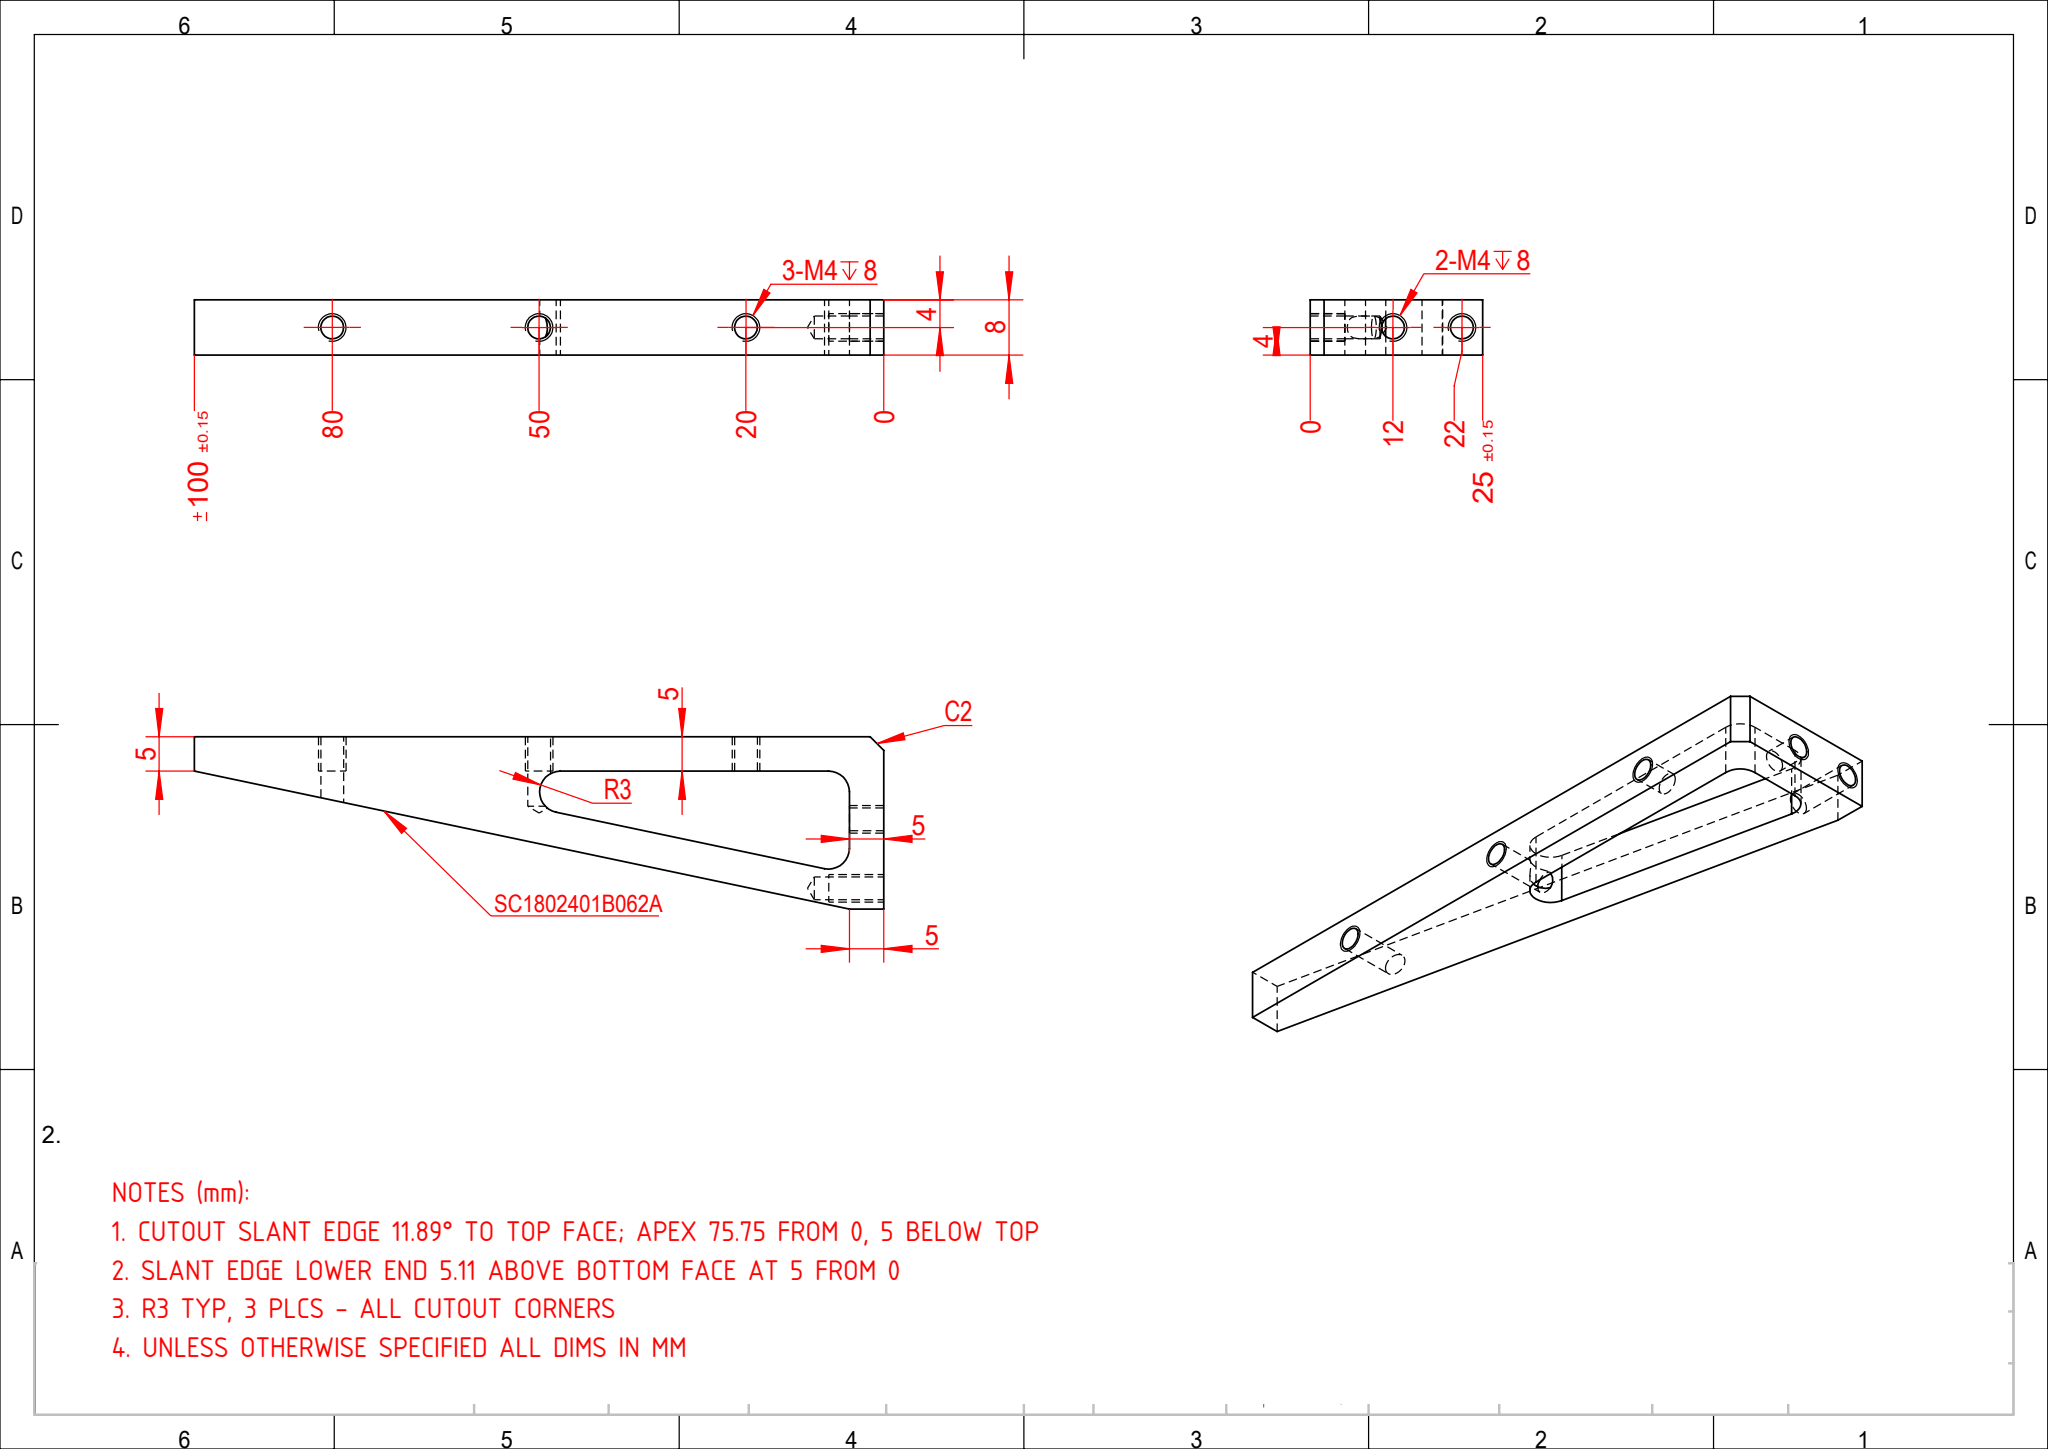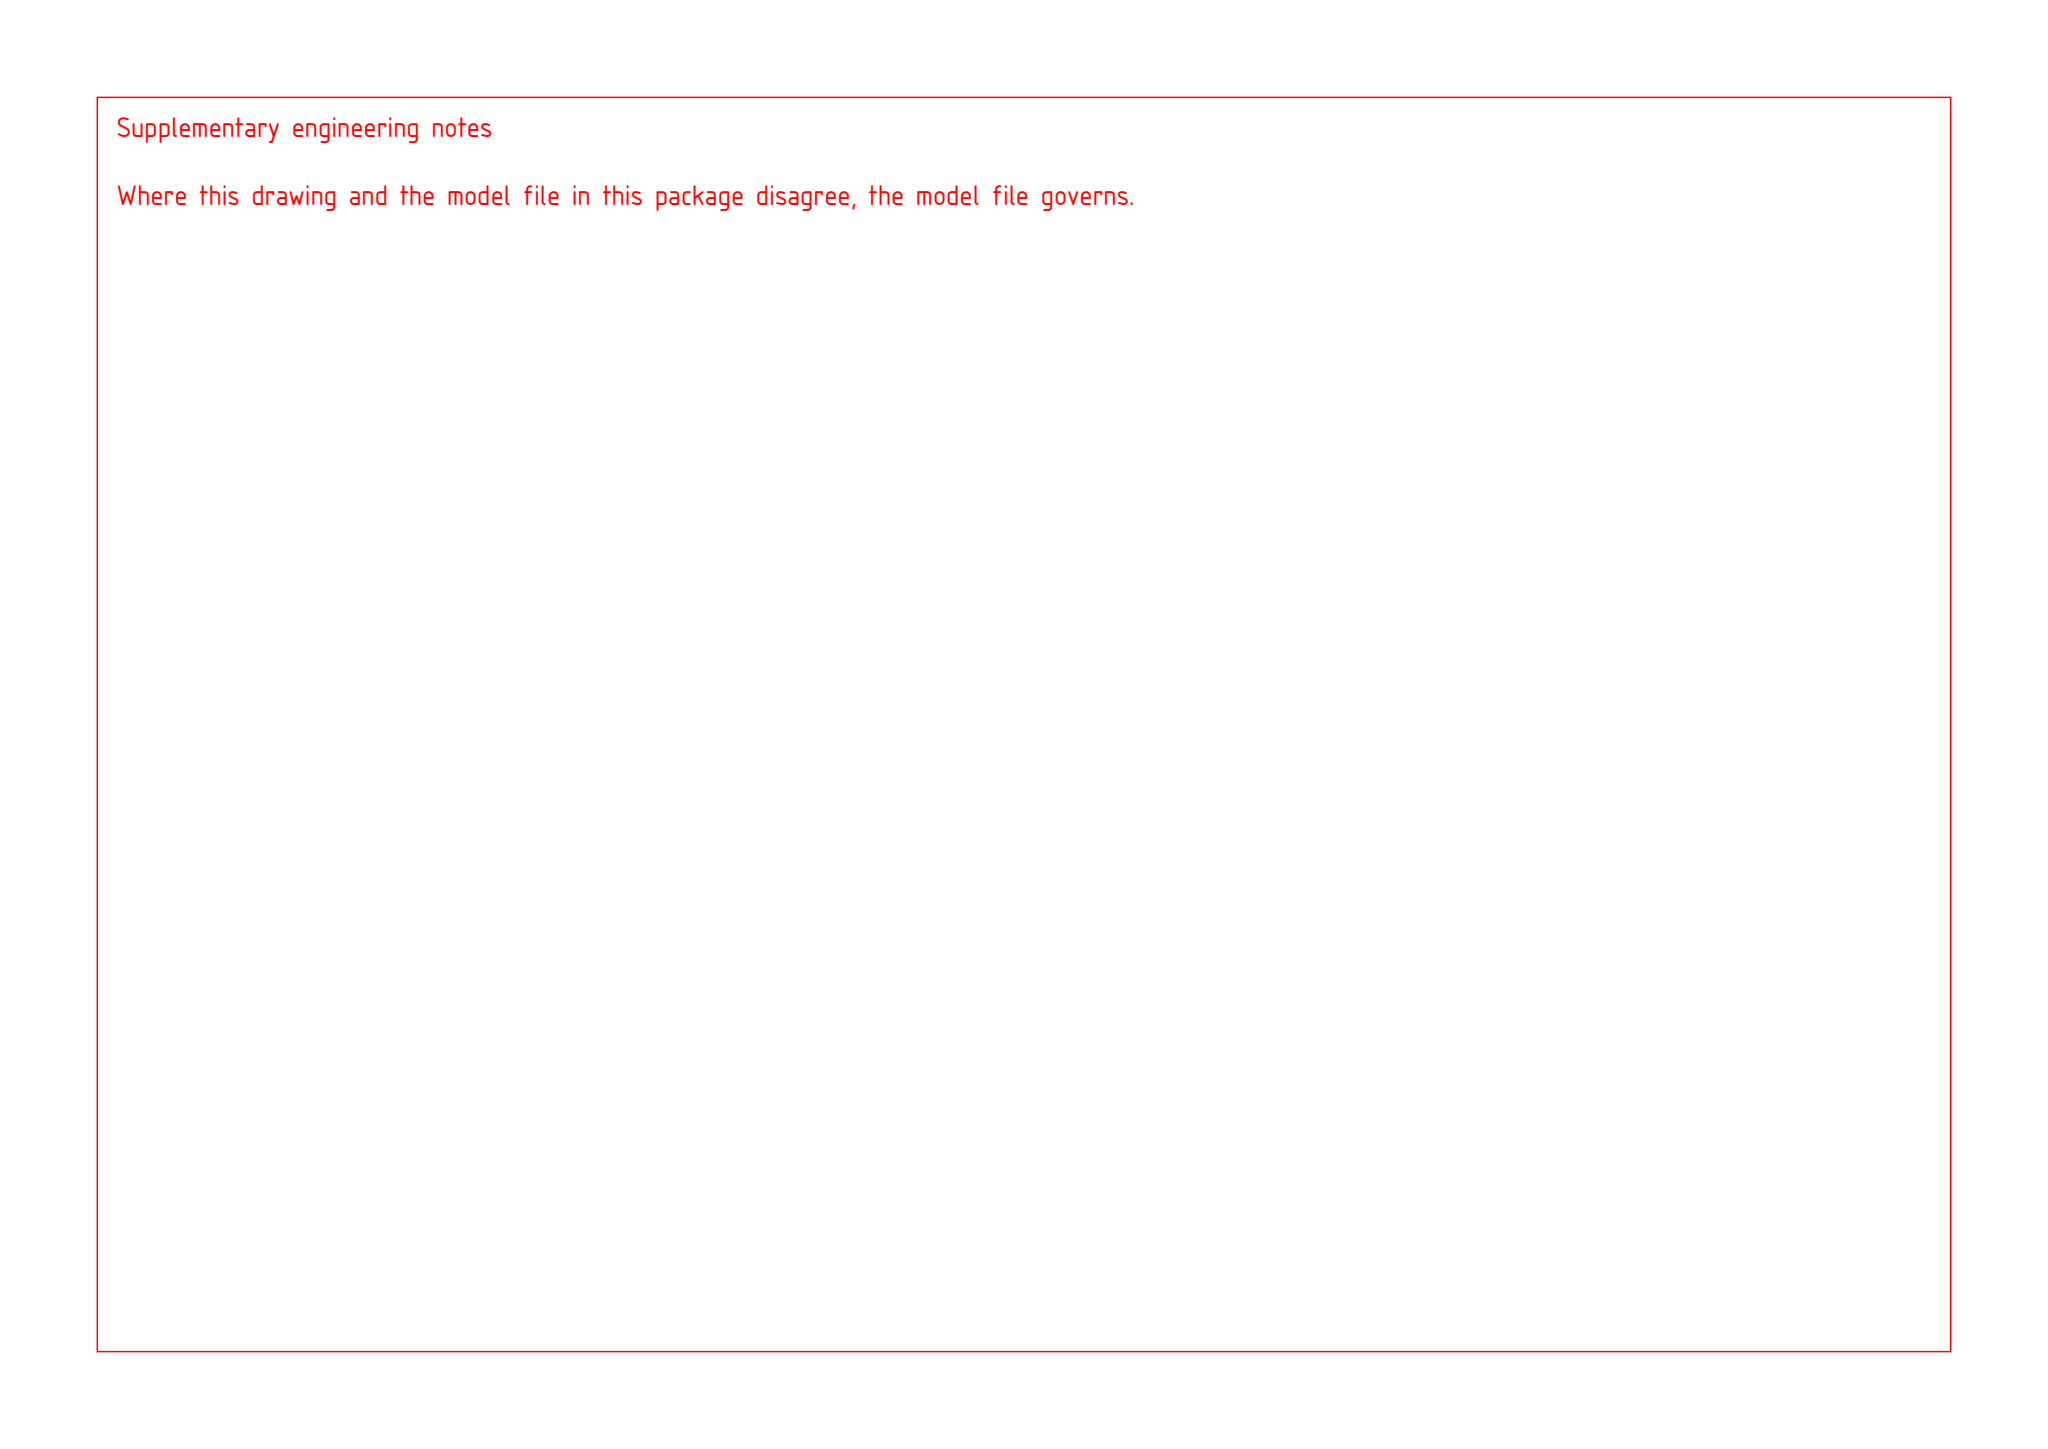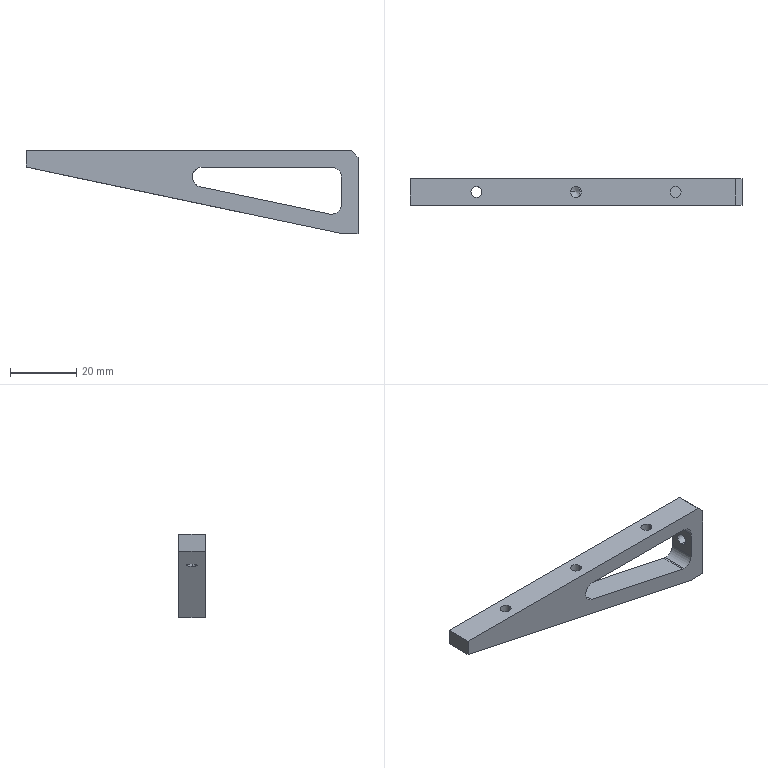Part | SolidWorks | mm | 1 solid | 29 faces | box 100 x 8 x 25 mm | volume 8468 mm3 | cylinder 14 | plane 11 | cone 4 | commonest cylinder face diameters 3.3 x10 6 x4
Drawing notes:
CUTOUT SLANT EDGE 11.89° TO TOP FACE; APEX 75.75 FROM 0, 5 BELOW TOP | from the solid: R3 corner centers (x,z)=(53.08,17) & (92,8.81) in STEP: slope 8.19/38.92 = 11.887 deg; tangent line z=25.104-0.2104x meets z=20 (5 below z=25 top) at x=24.26, i.e. 100-24.26=75.75 from the 0 end face
SLANT EDGE LOWER END 5.11 ABOVE BOTTOM FACE AT 5 FROM 0 | from the solid: Same tangent line at x=95 (vertical cutout wall, 5 from x=100 thick end face) gives z=5.11 above z=0 bottom plane
R3 TYP, 3 PLCS - ALL CUTOUT CORNERS | from the solid: Three Ø6.0 y-axis cylinders (full 8 thk) at (53.08,17), (92,17), (92,8.81) = R3 corner radii
UNLESS OTHERWISE SPECIFIED ALL DIMS IN MM | from the solid: STEP bbox 100.0 x 8.0 x 25.0 mm, M4 threads, R3